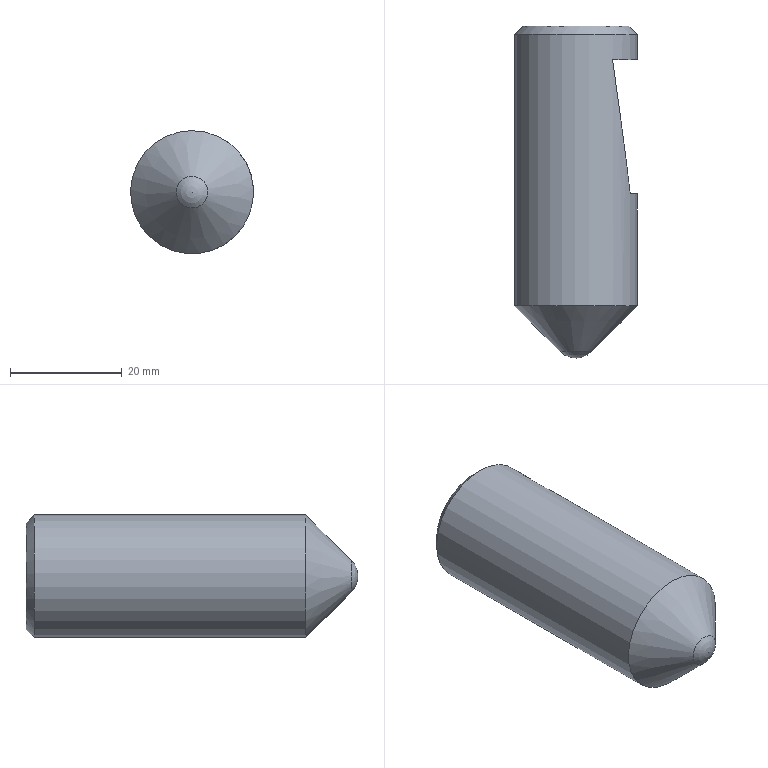Component | NX | LOCATING_SHAFT | 1 solid | 8 faces | box 22 x 59.34 x 22 mm | volume 18738 mm3 | plane 4 | cone 2 | cylinder 1 | sphere 1 | commonest cylinder face diameters 22 x1
STEP:
#1=CARTESIAN_POINT('',(0.,0.,0.));
#2=DIRECTION('',(0.,0.,1.));
#3=DIRECTION('',(1.,0.,0.));
#4=AXIS2_PLACEMENT_3D('',#1,#2,#3);
#5=CARTESIAN_POINT('',(-30.536,-43.411,2.847));
#6=VERTEX_POINT('',#5);
#7=CARTESIAN_POINT('',(-19.911,-43.411,-0.));
#8=DIRECTION('',(0.,-1.,0.));
#9=DIRECTION('',(-0.9659,0.,0.2588));
#10=AXIS2_PLACEMENT_3D('',#7,#8,#9);
#11=CIRCLE('',#10,11.);
#12=CARTESIAN_POINT('',(-19.911,-91.911,-0.));
#13=DIRECTION('',(0.,1.,0.));
#14=DIRECTION('',(-0.9659,0.,0.2588));
#15=AXIS2_PLACEMENT_3D('',#12,#13,#14);
#16=CYLINDRICAL_SURFACE('',#15,11.);
#17=CARTESIAN_POINT('',(6.283,48.5));
#18=DIRECTION('',(-1.,0.));
#19=VECTOR('',#18,1.);
#20=LINE('',#17,#19);
#21=(GEOMETRIC_REPRESENTATION_CONTEXT(2)PARAMETRIC_REPRESENTATION_CONTEXT()REPRESENTATION_CONTEXT('',''));
#22=DEFINITIONAL_REPRESENTATION('',(#20),#21);
#23=PCURVE('',#16,#22);
#24=CARTESIAN_POINT('',(-19.911,-41.911,-0.));
#25=DIRECTION('',(0.,-1.,0.));
#26=DIRECTION('',(0.9659,0.,-0.2588));
#27=AXIS2_PLACEMENT_3D('',#24,#25,#26);
#28=CONICAL_SURFACE('',#27,9.5,0.7854);
#29=CARTESIAN_POINT('',(3.142,1.5));
#30=DIRECTION('',(1.,0.));
#31=VECTOR('',#30,1.);
#32=LINE('',#29,#31);
#33=(GEOMETRIC_REPRESENTATION_CONTEXT(2)PARAMETRIC_REPRESENTATION_CONTEXT()REPRESENTATION_CONTEXT('',''));
#34=DEFINITIONAL_REPRESENTATION('',(#32),#33);
#35=PCURVE('',#28,#34);
#36=SURFACE_CURVE('',#11,(#23,#35),.PCURVE_S1.);
#37=EDGE_CURVE('',#6,#6,#36,.T.);
#38=ORIENTED_EDGE('',*,*,#37,.T.);
#39=CARTESIAN_POINT('',(-30.536,-91.911,2.847));
#40=VERTEX_POINT('',#39);
#41=CARTESIAN_POINT('',(-30.536,-91.911,2.847));
#42=CARTESIAN_POINT('',(-30.536,-43.411,2.847));
#43=B_SPLINE_CURVE_WITH_KNOTS('',1,(#41,#42),.UNSPECIFIED.,.F.,.F.,(2,2),(0.,48.5),.PIECEWISE_BEZIER_KNOTS.);
#44=CARTESIAN_POINT('',(0.,0.));
#45=DIRECTION('',(0.,1.));
#46=VECTOR('',#45,1.);
#47=LINE('',#44,#46);
#48=(GEOMETRIC_REPRESENTATION_CONTEXT(2)PARAMETRIC_REPRESENTATION_CONTEXT()REPRESENTATION_CONTEXT('',''));
#49=DEFINITIONAL_REPRESENTATION('',(#47),#48);
#50=PCURVE('',#16,#49);
#51=CARTESIAN_POINT('',(6.283,0.));
#52=DIRECTION('',(0.,1.));
#53=VECTOR('',#52,1.);
#54=LINE('',#51,#53);
#55=(GEOMETRIC_REPRESENTATION_CONTEXT(2)PARAMETRIC_REPRESENTATION_CONTEXT()REPRESENTATION_CONTEXT('',''));
#56=DEFINITIONAL_REPRESENTATION('',(#54),#55);
#57=PCURVE('',#16,#56);
#58=SEAM_CURVE('',#43,(#50,#57),.PCURVE_S1.);
#59=EDGE_CURVE('',#40,#6,#58,.T.);
#60=ORIENTED_EDGE('',*,*,#59,.F.);
#61=CARTESIAN_POINT('',(-19.911,-91.911,-0.));
#62=DIRECTION('',(0.,1.,0.));
#63=DIRECTION('',(-0.9659,0.,0.2588));
#64=AXIS2_PLACEMENT_3D('',#61,#62,#63);
#65=CIRCLE('',#64,11.);
#66=CARTESIAN_POINT('',(0.,0.));
#67=DIRECTION('',(1.,0.));
#68=VECTOR('',#67,1.);
#69=LINE('',#66,#68);
#70=(GEOMETRIC_REPRESENTATION_CONTEXT(2)PARAMETRIC_REPRESENTATION_CONTEXT()REPRESENTATION_CONTEXT('',''));
#71=DEFINITIONAL_REPRESENTATION('',(#69),#70);
#72=PCURVE('',#16,#71);
#73=CARTESIAN_POINT('',(-19.911,-91.911,-0.));
#74=DIRECTION('',(0.,1.,0.));
#75=DIRECTION('',(-0.9659,0.,0.2588));
#76=AXIS2_PLACEMENT_3D('',#73,#74,#75);
#77=CONICAL_SURFACE('',#76,11.,0.7854);
#78=CARTESIAN_POINT('',(0.,0.));
#79=DIRECTION('',(1.,0.));
#80=VECTOR('',#79,1.);
#81=LINE('',#78,#80);
#82=(GEOMETRIC_REPRESENTATION_CONTEXT(2)PARAMETRIC_REPRESENTATION_CONTEXT()REPRESENTATION_CONTEXT('',''));
#83=DEFINITIONAL_REPRESENTATION('',(#81),#82);
#84=PCURVE('',#77,#83);
#85=SURFACE_CURVE('',#65,(#72,#84),.PCURVE_S1.);
#86=EDGE_CURVE('',#40,#40,#85,.T.);
#87=ORIENTED_EDGE('',*,*,#86,.T.);
#88=ORIENTED_EDGE('',*,*,#59,.T.);
#89=EDGE_LOOP('',(#38,#60,#87,#88));
#90=FACE_BOUND('',#89,.T.);
#91=CARTESIAN_POINT('',(-13.395,-47.911,8.863));
#92=VERTEX_POINT('',#91);
#93=CARTESIAN_POINT('',(-18.699,-47.911,-10.933));
#94=VERTEX_POINT('',#93);
#95=CARTESIAN_POINT('',(-19.911,-47.911,-0.));
#96=DIRECTION('',(0.,1.,0.));
#97=DIRECTION('',(0.9659,0.,-0.2588));
#98=AXIS2_PLACEMENT_3D('',#95,#96,#97);
#99=CIRCLE('',#98,11.);
#100=CARTESIAN_POINT('',(-3.142,44.));
#101=DIRECTION('',(1.,0.));
#102=VECTOR('',#101,1.);
#103=LINE('',#100,#102);
#104=(GEOMETRIC_REPRESENTATION_CONTEXT(2)PARAMETRIC_REPRESENTATION_CONTEXT()REPRESENTATION_CONTEXT('',''));
#105=DEFINITIONAL_REPRESENTATION('',(#103),#104);
#106=PCURVE('',#16,#105);
#107=CARTESIAN_POINT('',(-28.988,-47.911,-49.332));
#108=DIRECTION('',(0.,-1.,0.));
#109=DIRECTION('',(0.9659,0.,-0.2588));
#110=AXIS2_PLACEMENT_3D('',#107,#108,#109);
#111=PLANE('',#110);
#112=CARTESIAN_POINT('',(7.,50.));
#113=CARTESIAN_POINT('',(7.,30.947));
#114=CARTESIAN_POINT('',(-9.5,40.474));
#115=CARTESIAN_POINT('',(-26.,50.));
#116=CARTESIAN_POINT('',(-9.5,59.526));
#117=CARTESIAN_POINT('',(7.,69.053));
#118=CARTESIAN_POINT('',(7.,50.));
#119=(BOUNDED_CURVE()B_SPLINE_CURVE(2,(#112,#113,#114,#115,#116,#117,#118),.UNSPECIFIED.,.T.,.F.)B_SPLINE_CURVE_WITH_KNOTS((1,2,2,2,2,1),(-2.094,0.,2.094,4.189,6.283,8.378),.UNSPECIFIED.)CURVE()GEOMETRIC_REPRESENTATION_ITEM()RATIONAL_B_SPLINE_CURVE((1.,0.5,1.,0.5,1.,0.5,1.))REPRESENTATION_ITEM(''));
#120=(GEOMETRIC_REPRESENTATION_CONTEXT(2)PARAMETRIC_REPRESENTATION_CONTEXT()REPRESENTATION_CONTEXT('',''));
#121=DEFINITIONAL_REPRESENTATION('',(#119),#120);
#122=PCURVE('',#111,#121);
#123=SURFACE_CURVE('',#99,(#106,#122),.PCURVE_S1.);
#124=EDGE_CURVE('',#92,#94,#123,.T.);
#125=ORIENTED_EDGE('',*,*,#124,.T.);
#126=CARTESIAN_POINT('',(-14.138,-71.911,-9.363));
#127=VERTEX_POINT('',#126);
#128=CARTESIAN_POINT('',(-19.911,-23.911,-0.));
#129=DIRECTION('',(-0.9528,-0.1644,0.2553));
#130=DIRECTION('',(-0.1588,0.9864,0.04255));
#131=AXIS2_PLACEMENT_3D('',#128,#129,#130);
#132=ELLIPSE('',#131,66.91,11.);
#133=CARTESIAN_POINT('',(4.34,44.));
#134=CARTESIAN_POINT('',(4.334,43.588));
#135=CARTESIAN_POINT('',(4.32,42.768));
#136=CARTESIAN_POINT('',(4.3,41.547));
#137=CARTESIAN_POINT('',(4.28,40.337));
#138=CARTESIAN_POINT('',(4.26,39.138));
#139=CARTESIAN_POINT('',(4.24,37.951));
#140=CARTESIAN_POINT('',(4.22,36.776));
#141=CARTESIAN_POINT('',(4.2,35.614));
#142=CARTESIAN_POINT('',(4.179,34.464));
#143=CARTESIAN_POINT('',(4.159,33.328));
#144=CARTESIAN_POINT('',(4.139,32.207));
#145=CARTESIAN_POINT('',(4.119,31.099));
#146=CARTESIAN_POINT('',(4.099,30.007));
#147=CARTESIAN_POINT('',(4.079,28.93));
#148=CARTESIAN_POINT('',(4.059,27.869));
#149=CARTESIAN_POINT('',(4.039,26.824));
#150=CARTESIAN_POINT('',(4.019,25.795));
#151=CARTESIAN_POINT('',(3.999,24.784));
#152=CARTESIAN_POINT('',(3.978,23.79));
#153=CARTESIAN_POINT('',(3.958,22.814));
#154=CARTESIAN_POINT('',(3.938,21.856));
#155=CARTESIAN_POINT('',(3.918,20.917));
#156=CARTESIAN_POINT('',(3.905,20.303));
#157=CARTESIAN_POINT('',(3.898,20.));
#158=B_SPLINE_CURVE_WITH_KNOTS('',3,(#133,#134,#135,#136,#137,#138,#139,#140,#141,#142,#143,#144,#145,#146,#147,#148,#149,#150,#151,#152,#153,#154,#155,#156,#157),.UNSPECIFIED.,.F.,.F.,(4,1,1,1,1,1,1,1,1,1,1,1,1,1,1,1,1,1,1,1,1,1,4),(1.943,1.963,1.983,2.003,2.023,2.043,2.064,2.084,2.104,2.124,2.144,2.164,2.184,2.204,2.224,2.244,2.265,2.285,2.305,2.325,2.345,2.365,2.385),.QUASI_UNIFORM_KNOTS.);
#159=(GEOMETRIC_REPRESENTATION_CONTEXT(2)PARAMETRIC_REPRESENTATION_CONTEXT()REPRESENTATION_CONTEXT('',''));
#160=DEFINITIONAL_REPRESENTATION('',(#158),#159);
#161=PCURVE('',#16,#160);
#162=CARTESIAN_POINT('',(-25.125,-71.911,-50.367));
#163=DIRECTION('',(0.9528,0.1644,-0.2553));
#164=DIRECTION('',(-0.1588,0.9864,0.04255));
#165=AXIS2_PLACEMENT_3D('',#162,#163,#164);
#166=PLANE('',#165);
#167=CARTESIAN_POINT('',(115.572,50.));
#168=CARTESIAN_POINT('',(115.572,30.947));
#169=CARTESIAN_POINT('',(15.207,40.474));
#170=CARTESIAN_POINT('',(-85.159,50.));
#171=CARTESIAN_POINT('',(15.207,59.526));
#172=CARTESIAN_POINT('',(115.572,69.053));
#173=CARTESIAN_POINT('',(115.572,50.));
#174=(BOUNDED_CURVE()B_SPLINE_CURVE(2,(#167,#168,#169,#170,#171,#172,#173),.UNSPECIFIED.,.T.,.F.)B_SPLINE_CURVE_WITH_KNOTS((1,2,2,2,2,1),(-2.094,0.,2.094,4.189,6.283,8.378),.UNSPECIFIED.)CURVE()GEOMETRIC_REPRESENTATION_ITEM()RATIONAL_B_SPLINE_CURVE((1.,0.5,1.,0.5,1.,0.5,1.))REPRESENTATION_ITEM(''));
#175=(GEOMETRIC_REPRESENTATION_CONTEXT(2)PARAMETRIC_REPRESENTATION_CONTEXT()REPRESENTATION_CONTEXT('',''));
#176=DEFINITIONAL_REPRESENTATION('',(#174),#175);
#177=PCURVE('',#166,#176);
#178=SURFACE_CURVE('',#132,(#161,#177),.PCURVE_S1.);
#179=EDGE_CURVE('',#94,#127,#178,.T.);
#180=ORIENTED_EDGE('',*,*,#179,.T.);
#181=CARTESIAN_POINT('',(-10.23,-71.911,5.222));
#182=VERTEX_POINT('',#181);
#183=CARTESIAN_POINT('',(-19.911,-71.911,-0.));
#184=DIRECTION('',(0.,-1.,0.));
#185=DIRECTION('',(-0.9659,0.,0.2588));
#186=AXIS2_PLACEMENT_3D('',#183,#184,#185);
#187=CIRCLE('',#186,11.);
#188=CARTESIAN_POINT('',(6.283,20.));
#189=DIRECTION('',(-1.,0.));
#190=VECTOR('',#189,1.);
#191=LINE('',#188,#190);
#192=(GEOMETRIC_REPRESENTATION_CONTEXT(2)PARAMETRIC_REPRESENTATION_CONTEXT()REPRESENTATION_CONTEXT('',''));
#193=DEFINITIONAL_REPRESENTATION('',(#191),#192);
#194=PCURVE('',#16,#193);
#195=CARTESIAN_POINT('',(-22.227,-71.911,-51.143));
#196=DIRECTION('',(0.,1.,0.));
#197=DIRECTION('',(-0.9659,0.,0.2588));
#198=AXIS2_PLACEMENT_3D('',#195,#196,#197);
#199=PLANE('',#198);
#200=CARTESIAN_POINT('',(22.,50.));
#201=CARTESIAN_POINT('',(22.,30.947));
#202=CARTESIAN_POINT('',(5.5,40.474));
#203=CARTESIAN_POINT('',(-11.,50.));
#204=CARTESIAN_POINT('',(5.5,59.526));
#205=CARTESIAN_POINT('',(22.,69.053));
#206=CARTESIAN_POINT('',(22.,50.));
#207=(BOUNDED_CURVE()B_SPLINE_CURVE(2,(#200,#201,#202,#203,#204,#205,#206),.UNSPECIFIED.,.T.,.F.)B_SPLINE_CURVE_WITH_KNOTS((1,2,2,2,2,1),(-2.094,0.,2.094,4.189,6.283,8.378),.UNSPECIFIED.)CURVE()GEOMETRIC_REPRESENTATION_ITEM()RATIONAL_B_SPLINE_CURVE((1.,0.5,1.,0.5,1.,0.5,1.))REPRESENTATION_ITEM(''));
#208=(GEOMETRIC_REPRESENTATION_CONTEXT(2)PARAMETRIC_REPRESENTATION_CONTEXT()REPRESENTATION_CONTEXT('',''));
#209=DEFINITIONAL_REPRESENTATION('',(#207),#208);
#210=PCURVE('',#199,#209);
#211=SURFACE_CURVE('',#187,(#194,#210),.PCURVE_S1.);
#212=EDGE_CURVE('',#127,#182,#211,.T.);
#213=ORIENTED_EDGE('',*,*,#212,.T.);
#214=CARTESIAN_POINT('',(-19.911,-23.911,-0.));
#215=DIRECTION('',(-0.9528,-0.1644,0.2553));
#216=DIRECTION('',(-0.1588,0.9864,0.04255));
#217=AXIS2_PLACEMENT_3D('',#214,#215,#216);
#218=ELLIPSE('',#217,66.91,11.);
#219=CARTESIAN_POINT('',(2.385,20.));
#220=CARTESIAN_POINT('',(2.378,20.303));
#221=CARTESIAN_POINT('',(2.365,20.917));
#222=CARTESIAN_POINT('',(2.345,21.856));
#223=CARTESIAN_POINT('',(2.325,22.814));
#224=CARTESIAN_POINT('',(2.305,23.79));
#225=CARTESIAN_POINT('',(2.285,24.784));
#226=CARTESIAN_POINT('',(2.265,25.795));
#227=CARTESIAN_POINT('',(2.244,26.824));
#228=CARTESIAN_POINT('',(2.224,27.869));
#229=CARTESIAN_POINT('',(2.204,28.93));
#230=CARTESIAN_POINT('',(2.184,30.007));
#231=CARTESIAN_POINT('',(2.164,31.099));
#232=CARTESIAN_POINT('',(2.144,32.207));
#233=CARTESIAN_POINT('',(2.124,33.328));
#234=CARTESIAN_POINT('',(2.104,34.464));
#235=CARTESIAN_POINT('',(2.084,35.614));
#236=CARTESIAN_POINT('',(2.064,36.776));
#237=CARTESIAN_POINT('',(2.043,37.951));
#238=CARTESIAN_POINT('',(2.023,39.138));
#239=CARTESIAN_POINT('',(2.003,40.337));
#240=CARTESIAN_POINT('',(1.983,41.547));
#241=CARTESIAN_POINT('',(1.963,42.768));
#242=CARTESIAN_POINT('',(1.95,43.588));
#243=CARTESIAN_POINT('',(1.943,44.));
#244=B_SPLINE_CURVE_WITH_KNOTS('',3,(#219,#220,#221,#222,#223,#224,#225,#226,#227,#228,#229,#230,#231,#232,#233,#234,#235,#236,#237,#238,#239,#240,#241,#242,#243),.UNSPECIFIED.,.F.,.F.,(4,1,1,1,1,1,1,1,1,1,1,1,1,1,1,1,1,1,1,1,1,1,4),(3.898,3.918,3.938,3.958,3.978,3.999,4.019,4.039,4.059,4.079,4.099,4.119,4.139,4.159,4.179,4.2,4.22,4.24,4.26,4.28,4.3,4.32,4.34),.QUASI_UNIFORM_KNOTS.);
#245=(GEOMETRIC_REPRESENTATION_CONTEXT(2)PARAMETRIC_REPRESENTATION_CONTEXT()REPRESENTATION_CONTEXT('',''));
#246=DEFINITIONAL_REPRESENTATION('',(#244),#245);
#247=PCURVE('',#16,#246);
#248=CARTESIAN_POINT('',(115.572,50.));
#249=CARTESIAN_POINT('',(115.572,30.947));
#250=CARTESIAN_POINT('',(15.207,40.474));
#251=CARTESIAN_POINT('',(-85.159,50.));
#252=CARTESIAN_POINT('',(15.207,59.526));
#253=CARTESIAN_POINT('',(115.572,69.053));
#254=CARTESIAN_POINT('',(115.572,50.));
#255=(BOUNDED_CURVE()B_SPLINE_CURVE(2,(#248,#249,#250,#251,#252,#253,#254),.UNSPECIFIED.,.T.,.F.)B_SPLINE_CURVE_WITH_KNOTS((1,2,2,2,2,1),(-2.094,0.,2.094,4.189,6.283,8.378),.UNSPECIFIED.)CURVE()GEOMETRIC_REPRESENTATION_ITEM()RATIONAL_B_SPLINE_CURVE((1.,0.5,1.,0.5,1.,0.5,1.))REPRESENTATION_ITEM(''));
#256=(GEOMETRIC_REPRESENTATION_CONTEXT(2)PARAMETRIC_REPRESENTATION_CONTEXT()REPRESENTATION_CONTEXT('',''));
#257=DEFINITIONAL_REPRESENTATION('',(#255),#256);
#258=PCURVE('',#166,#257);
#259=SURFACE_CURVE('',#218,(#247,#258),.PCURVE_S1.);
#260=EDGE_CURVE('',#182,#92,#259,.T.);
#261=ORIENTED_EDGE('',*,*,#260,.T.);
#262=EDGE_LOOP('',(#125,#180,#213,#261));
#263=FACE_BOUND('',#262,.T.);
#264=ADVANCED_FACE('',(#90,#263),#16,.T.);
#265=CARTESIAN_POINT('',(-29.087,-41.911,2.459));
#266=VERTEX_POINT('',#265);
#267=CARTESIAN_POINT('',(-19.911,-41.911,-0.));
#268=DIRECTION('',(0.,1.,0.));
#269=DIRECTION('',(-0.9659,0.,0.2588));
#270=AXIS2_PLACEMENT_3D('',#267,#268,#269);
#271=CIRCLE('',#270,9.5);
#272=CARTESIAN_POINT('',(-19.911,-41.911,-0.));
#273=DIRECTION('',(0.,1.,0.));
#274=DIRECTION('',(-0.9659,0.,0.2588));
#275=AXIS2_PLACEMENT_3D('',#272,#273,#274);
#276=PLANE('',#275);
#277=CARTESIAN_POINT('',(0.,0.));
#278=DIRECTION('',(1.,0.));
#279=AXIS2_PLACEMENT_2D('',#277,#278);
#280=CIRCLE('',#279,9.5);
#281=(GEOMETRIC_REPRESENTATION_CONTEXT(2)PARAMETRIC_REPRESENTATION_CONTEXT()REPRESENTATION_CONTEXT('',''));
#282=DEFINITIONAL_REPRESENTATION('',(#280),#281);
#283=PCURVE('',#276,#282);
#284=CARTESIAN_POINT('',(9.425,-0.));
#285=DIRECTION('',(-1.,0.));
#286=VECTOR('',#285,1.);
#287=LINE('',#284,#286);
#288=(GEOMETRIC_REPRESENTATION_CONTEXT(2)PARAMETRIC_REPRESENTATION_CONTEXT()REPRESENTATION_CONTEXT('',''));
#289=DEFINITIONAL_REPRESENTATION('',(#287),#288);
#290=PCURVE('',#28,#289);
#291=SURFACE_CURVE('',#271,(#283,#290),.PCURVE_S1.);
#292=EDGE_CURVE('',#266,#266,#291,.T.);
#293=ORIENTED_EDGE('',*,*,#292,.T.);
#294=EDGE_LOOP('',(#293));
#295=FACE_BOUND('',#294,.T.);
#296=ADVANCED_FACE('',(#295),#276,.T.);
#297=CARTESIAN_POINT('',(-22.643,-100.083,0.7321));
#298=VERTEX_POINT('',#297);
#299=CARTESIAN_POINT('',(-17.179,-100.083,-0.7321));
#300=VERTEX_POINT('',#299);
#301=CARTESIAN_POINT('',(-19.911,-100.083,-0.));
#302=DIRECTION('',(0.,1.,0.));
#303=DIRECTION('',(-0.9659,0.,0.2588));
#304=AXIS2_PLACEMENT_3D('',#301,#302,#303);
#305=CIRCLE('',#304,2.828);
#306=CARTESIAN_POINT('',(0.,-8.172));
#307=DIRECTION('',(1.,0.));
#308=VECTOR('',#307,1.);
#309=LINE('',#306,#308);
#310=(GEOMETRIC_REPRESENTATION_CONTEXT(2)PARAMETRIC_REPRESENTATION_CONTEXT()REPRESENTATION_CONTEXT('',''));
#311=DEFINITIONAL_REPRESENTATION('',(#309),#310);
#312=PCURVE('',#77,#311);
#313=CARTESIAN_POINT('',(-19.911,-97.254,-0.));
#314=DIRECTION('',(0.,1.,-0.));
#315=DIRECTION('',(0.9659,-0.,-0.2588));
#316=AXIS2_PLACEMENT_3D('',#313,#314,#315);
#317=SPHERICAL_SURFACE('',#316,4.);
#318=CARTESIAN_POINT('',(3.142,-0.7854));
#319=CARTESIAN_POINT('',(3.237,-0.7854));
#320=CARTESIAN_POINT('',(3.427,-0.7854));
#321=CARTESIAN_POINT('',(3.713,-0.7854));
#322=CARTESIAN_POINT('',(3.998,-0.7854));
#323=CARTESIAN_POINT('',(4.284,-0.7854));
#324=CARTESIAN_POINT('',(4.57,-0.7854));
#325=CARTESIAN_POINT('',(4.855,-0.7854));
#326=CARTESIAN_POINT('',(5.141,-0.7854));
#327=CARTESIAN_POINT('',(5.426,-0.7854));
#328=CARTESIAN_POINT('',(5.712,-0.7854));
#329=CARTESIAN_POINT('',(5.998,-0.7854));
#330=CARTESIAN_POINT('',(6.283,-0.7854));
#331=CARTESIAN_POINT('',(6.569,-0.7854));
#332=CARTESIAN_POINT('',(6.854,-0.7854));
#333=CARTESIAN_POINT('',(7.14,-0.7854));
#334=CARTESIAN_POINT('',(7.426,-0.7854));
#335=CARTESIAN_POINT('',(7.711,-0.7854));
#336=CARTESIAN_POINT('',(7.997,-0.7854));
#337=CARTESIAN_POINT('',(8.282,-0.7854));
#338=CARTESIAN_POINT('',(8.568,-0.7854));
#339=CARTESIAN_POINT('',(8.854,-0.7854));
#340=CARTESIAN_POINT('',(9.139,-0.7854));
#341=CARTESIAN_POINT('',(9.33,-0.7854));
#342=CARTESIAN_POINT('',(9.425,-0.7854));
#343=B_SPLINE_CURVE_WITH_KNOTS('',3,(#318,#319,#320,#321,#322,#323,#324,#325,#326,#327,#328,#329,#330,#331,#332,#333,#334,#335,#336,#337,#338,#339,#340,#341,#342),.UNSPECIFIED.,.F.,.F.,(4,1,1,1,1,1,1,1,1,1,1,1,1,1,1,1,1,1,1,1,1,1,4),(0.,0.2856,0.5712,0.8568,1.142,1.428,1.714,1.999,2.285,2.57,2.856,3.142,3.427,3.713,3.998,4.284,4.57,4.855,5.141,5.426,5.712,5.998,6.283),.QUASI_UNIFORM_KNOTS.);
#344=(GEOMETRIC_REPRESENTATION_CONTEXT(2)PARAMETRIC_REPRESENTATION_CONTEXT()REPRESENTATION_CONTEXT('',''));
#345=DEFINITIONAL_REPRESENTATION('',(#343),#344);
#346=PCURVE('',#317,#345);
#347=SURFACE_CURVE('',#305,(#312,#346),.PCURVE_S1.);
#348=EDGE_CURVE('',#298,#300,#347,.T.);
#349=ORIENTED_EDGE('',*,*,#348,.T.);
#350=CARTESIAN_POINT('',(-19.911,-100.083,-0.));
#351=DIRECTION('',(0.,1.,0.));
#352=DIRECTION('',(-0.9659,0.,0.2588));
#353=AXIS2_PLACEMENT_3D('',#350,#351,#352);
#354=CIRCLE('',#353,2.828);
#355=CARTESIAN_POINT('',(0.,-8.172));
#356=DIRECTION('',(1.,0.));
#357=VECTOR('',#356,1.);
#358=LINE('',#355,#357);
#359=(GEOMETRIC_REPRESENTATION_CONTEXT(2)PARAMETRIC_REPRESENTATION_CONTEXT()REPRESENTATION_CONTEXT('',''));
#360=DEFINITIONAL_REPRESENTATION('',(#358),#359);
#361=PCURVE('',#77,#360);
#362=CARTESIAN_POINT('',(-3.142,-0.7854));
#363=CARTESIAN_POINT('',(-3.046,-0.7854));
#364=CARTESIAN_POINT('',(-2.856,-0.7854));
#365=CARTESIAN_POINT('',(-2.57,-0.7854));
#366=CARTESIAN_POINT('',(-2.285,-0.7854));
#367=CARTESIAN_POINT('',(-1.999,-0.7854));
#368=CARTESIAN_POINT('',(-1.714,-0.7854));
#369=CARTESIAN_POINT('',(-1.428,-0.7854));
#370=CARTESIAN_POINT('',(-1.142,-0.7854));
#371=CARTESIAN_POINT('',(-0.8568,-0.7854));
#372=CARTESIAN_POINT('',(-0.5712,-0.7854));
#373=CARTESIAN_POINT('',(-0.2856,-0.7854));
#374=CARTESIAN_POINT('',(-0.,-0.7854));
#375=CARTESIAN_POINT('',(0.2856,-0.7854));
#376=CARTESIAN_POINT('',(0.5712,-0.7854));
#377=CARTESIAN_POINT('',(0.8568,-0.7854));
#378=CARTESIAN_POINT('',(1.142,-0.7854));
#379=CARTESIAN_POINT('',(1.428,-0.7854));
#380=CARTESIAN_POINT('',(1.714,-0.7854));
#381=CARTESIAN_POINT('',(1.999,-0.7854));
#382=CARTESIAN_POINT('',(2.285,-0.7854));
#383=CARTESIAN_POINT('',(2.57,-0.7854));
#384=CARTESIAN_POINT('',(2.856,-0.7854));
#385=CARTESIAN_POINT('',(3.046,-0.7854));
#386=CARTESIAN_POINT('',(3.142,-0.7854));
#387=B_SPLINE_CURVE_WITH_KNOTS('',3,(#362,#363,#364,#365,#366,#367,#368,#369,#370,#371,#372,#373,#374,#375,#376,#377,#378,#379,#380,#381,#382,#383,#384,#385,#386),.UNSPECIFIED.,.F.,.F.,(4,1,1,1,1,1,1,1,1,1,1,1,1,1,1,1,1,1,1,1,1,1,4),(0.,0.2856,0.5712,0.8568,1.142,1.428,1.714,1.999,2.285,2.57,2.856,3.142,3.427,3.713,3.998,4.284,4.57,4.855,5.141,5.426,5.712,5.998,6.283),.QUASI_UNIFORM_KNOTS.);
#388=(GEOMETRIC_REPRESENTATION_CONTEXT(2)PARAMETRIC_REPRESENTATION_CONTEXT()REPRESENTATION_CONTEXT('',''));
#389=DEFINITIONAL_REPRESENTATION('',(#387),#388);
#390=PCURVE('',#317,#389);
#391=SURFACE_CURVE('',#354,(#361,#390),.PCURVE_S1.);
#392=EDGE_CURVE('',#300,#298,#391,.T.);
#393=ORIENTED_EDGE('',*,*,#392,.T.);
#394=CARTESIAN_POINT('',(-22.643,-100.083,0.7321));
#395=CARTESIAN_POINT('',(-30.536,-91.911,2.847));
#396=B_SPLINE_CURVE_WITH_KNOTS('',1,(#394,#395),.UNSPECIFIED.,.F.,.F.,(2,2),(-11.556,0.),.PIECEWISE_BEZIER_KNOTS.);
#397=CARTESIAN_POINT('',(6.283,0.));
#398=DIRECTION('',(0.,1.));
#399=VECTOR('',#398,1.);
#400=LINE('',#397,#399);
#401=(GEOMETRIC_REPRESENTATION_CONTEXT(2)PARAMETRIC_REPRESENTATION_CONTEXT()REPRESENTATION_CONTEXT('',''));
#402=DEFINITIONAL_REPRESENTATION('',(#400),#401);
#403=PCURVE('',#77,#402);
#404=CARTESIAN_POINT('',(0.,0.));
#405=DIRECTION('',(0.,1.));
#406=VECTOR('',#405,1.);
#407=LINE('',#404,#406);
#408=(GEOMETRIC_REPRESENTATION_CONTEXT(2)PARAMETRIC_REPRESENTATION_CONTEXT()REPRESENTATION_CONTEXT('',''));
#409=DEFINITIONAL_REPRESENTATION('',(#407),#408);
#410=PCURVE('',#77,#409);
#411=SEAM_CURVE('',#396,(#403,#410),.PCURVE_S1.);
#412=EDGE_CURVE('',#298,#40,#411,.T.);
#413=ORIENTED_EDGE('',*,*,#412,.T.);
#414=ORIENTED_EDGE('',*,*,#86,.F.);
#415=ORIENTED_EDGE('',*,*,#412,.F.);
#416=EDGE_LOOP('',(#349,#393,#413,#414,#415));
#417=FACE_BOUND('',#416,.T.);
#418=ADVANCED_FACE('',(#417),#77,.T.);
#419=ORIENTED_EDGE('',*,*,#392,.F.);
#420=CARTESIAN_POINT('',(-19.911,-101.254,-0.));
#421=VERTEX_POINT('',#420);
#422=CARTESIAN_POINT('',(-19.911,-101.254,-0.));
#423=CARTESIAN_POINT('',(-19.304,-101.254,-0.1626));
#424=CARTESIAN_POINT('',(-18.697,-101.131,-0.3252));
#425=CARTESIAN_POINT('',(-18.122,-100.884,-0.4795));
#426=CARTESIAN_POINT('',(-17.608,-100.527,-0.6171));
#427=CARTESIAN_POINT('',(-17.179,-100.083,-0.7321));
#428=B_SPLINE_CURVE_WITH_KNOTS('',5,(#422,#423,#424,#425,#426,#427),.UNSPECIFIED.,.F.,.F.,(6,6),(-1.571,-0.7854),.PIECEWISE_BEZIER_KNOTS.);
#429=CARTESIAN_POINT('',(0.,0.));
#430=DIRECTION('',(0.,1.));
#431=VECTOR('',#430,1.);
#432=LINE('',#429,#431);
#433=(GEOMETRIC_REPRESENTATION_CONTEXT(2)PARAMETRIC_REPRESENTATION_CONTEXT()REPRESENTATION_CONTEXT('',''));
#434=DEFINITIONAL_REPRESENTATION('',(#432),#433);
#435=PCURVE('',#317,#434);
#436=CARTESIAN_POINT('',(6.283,0.));
#437=DIRECTION('',(0.,1.));
#438=VECTOR('',#437,1.);
#439=LINE('',#436,#438);
#440=(GEOMETRIC_REPRESENTATION_CONTEXT(2)PARAMETRIC_REPRESENTATION_CONTEXT()REPRESENTATION_CONTEXT('',''));
#441=DEFINITIONAL_REPRESENTATION('',(#439),#440);
#442=PCURVE('',#317,#441);
#443=SEAM_CURVE('',#428,(#435,#442),.PCURVE_S1.);
#444=EDGE_CURVE('',#421,#300,#443,.T.);
#445=ORIENTED_EDGE('',*,*,#444,.F.);
#446=ORIENTED_EDGE('',*,*,#444,.T.);
#447=ORIENTED_EDGE('',*,*,#348,.F.);
#448=EDGE_LOOP('',(#419,#445,#446,#447));
#449=FACE_BOUND('',#448,.T.);
#450=ADVANCED_FACE('',(#449),#317,.T.);
#451=CARTESIAN_POINT('',(-25.125,-71.911,-50.367));
#452=DIRECTION('',(-0.2588,0.,-0.9659));
#453=VECTOR('',#452,1.);
#454=LINE('',#451,#453);
#455=CARTESIAN_POINT('',(3.,0.));
#456=DIRECTION('',(0.,-1.));
#457=VECTOR('',#456,1.);
#458=LINE('',#455,#457);
#459=(GEOMETRIC_REPRESENTATION_CONTEXT(2)PARAMETRIC_REPRESENTATION_CONTEXT()REPRESENTATION_CONTEXT('',''));
#460=DEFINITIONAL_REPRESENTATION('',(#458),#459);
#461=PCURVE('',#199,#460);
#462=CARTESIAN_POINT('',(0.,0.));
#463=DIRECTION('',(-0.,-1.));
#464=VECTOR('',#463,1.);
#465=LINE('',#462,#464);
#466=(GEOMETRIC_REPRESENTATION_CONTEXT(2)PARAMETRIC_REPRESENTATION_CONTEXT()REPRESENTATION_CONTEXT('',''));
#467=DEFINITIONAL_REPRESENTATION('',(#465),#466);
#468=PCURVE('',#166,#467);
#469=SURFACE_CURVE('',#454,(#461,#468),.PCURVE_S1.);
#470=EDGE_CURVE('',#182,#127,#469,.T.);
#471=ORIENTED_EDGE('',*,*,#470,.F.);
#472=ORIENTED_EDGE('',*,*,#212,.F.);
#473=EDGE_LOOP('',(#471,#472));
#474=FACE_BOUND('',#473,.T.);
#475=ADVANCED_FACE('',(#474),#199,.T.);
#476=CARTESIAN_POINT('',(-28.988,-47.911,-49.332));
#477=DIRECTION('',(-0.2588,0.,-0.9659));
#478=VECTOR('',#477,1.);
#479=LINE('',#476,#478);
#480=CARTESIAN_POINT('',(24.331,0.));
#481=DIRECTION('',(-0.,-1.));
#482=VECTOR('',#481,1.);
#483=LINE('',#480,#482);
#484=(GEOMETRIC_REPRESENTATION_CONTEXT(2)PARAMETRIC_REPRESENTATION_CONTEXT()REPRESENTATION_CONTEXT('',''));
#485=DEFINITIONAL_REPRESENTATION('',(#483),#484);
#486=PCURVE('',#166,#485);
#487=CARTESIAN_POINT('',(0.,0.));
#488=DIRECTION('',(0.,-1.));
#489=VECTOR('',#488,1.);
#490=LINE('',#487,#489);
#491=(GEOMETRIC_REPRESENTATION_CONTEXT(2)PARAMETRIC_REPRESENTATION_CONTEXT()REPRESENTATION_CONTEXT('',''));
#492=DEFINITIONAL_REPRESENTATION('',(#490),#491);
#493=PCURVE('',#111,#492);
#494=SURFACE_CURVE('',#479,(#486,#493),.PCURVE_S1.);
#495=EDGE_CURVE('',#92,#94,#494,.T.);
#496=ORIENTED_EDGE('',*,*,#495,.F.);
#497=ORIENTED_EDGE('',*,*,#260,.F.);
#498=ORIENTED_EDGE('',*,*,#470,.T.);
#499=ORIENTED_EDGE('',*,*,#179,.F.);
#500=EDGE_LOOP('',(#496,#497,#498,#499));
#501=FACE_BOUND('',#500,.T.);
#502=ADVANCED_FACE('',(#501),#166,.T.);
#503=ORIENTED_EDGE('',*,*,#124,.F.);
#504=ORIENTED_EDGE('',*,*,#495,.T.);
#505=EDGE_LOOP('',(#503,#504));
#506=FACE_BOUND('',#505,.T.);
#507=ADVANCED_FACE('',(#506),#111,.T.);
#508=ORIENTED_EDGE('',*,*,#37,.F.);
#509=CARTESIAN_POINT('',(-29.087,-41.911,2.459));
#510=CARTESIAN_POINT('',(-30.536,-43.411,2.847));
#511=B_SPLINE_CURVE_WITH_KNOTS('',1,(#509,#510),.UNSPECIFIED.,.F.,.F.,(2,2),(-0.,2.121),.PIECEWISE_BEZIER_KNOTS.);
#512=CARTESIAN_POINT('',(3.142,0.));
#513=DIRECTION('',(0.,1.));
#514=VECTOR('',#513,1.);
#515=LINE('',#512,#514);
#516=(GEOMETRIC_REPRESENTATION_CONTEXT(2)PARAMETRIC_REPRESENTATION_CONTEXT()REPRESENTATION_CONTEXT('',''));
#517=DEFINITIONAL_REPRESENTATION('',(#515),#516);
#518=PCURVE('',#28,#517);
#519=CARTESIAN_POINT('',(9.425,0.));
#520=DIRECTION('',(0.,1.));
#521=VECTOR('',#520,1.);
#522=LINE('',#519,#521);
#523=(GEOMETRIC_REPRESENTATION_CONTEXT(2)PARAMETRIC_REPRESENTATION_CONTEXT()REPRESENTATION_CONTEXT('',''));
#524=DEFINITIONAL_REPRESENTATION('',(#522),#523);
#525=PCURVE('',#28,#524);
#526=SEAM_CURVE('',#511,(#518,#525),.PCURVE_S1.);
#527=EDGE_CURVE('',#266,#6,#526,.T.);
#528=ORIENTED_EDGE('',*,*,#527,.F.);
#529=ORIENTED_EDGE('',*,*,#292,.F.);
#530=ORIENTED_EDGE('',*,*,#527,.T.);
#531=EDGE_LOOP('',(#508,#528,#529,#530));
#532=FACE_BOUND('',#531,.T.);
#533=ADVANCED_FACE('',(#532),#28,.T.);
#534=CLOSED_SHELL('',(#264,#296,#418,#450,#475,#502,#507,#533));
#535=MANIFOLD_SOLID_BREP('',#534);
#536=(LENGTH_UNIT()NAMED_UNIT(*)SI_UNIT(.MILLI.,.METRE.));
#537=UNCERTAINTY_MEASURE_WITH_UNIT(LENGTH_MEASURE(0.000005),#536,'','');
#538=(NAMED_UNIT(*)PLANE_ANGLE_UNIT()SI_UNIT($,.RADIAN.));
#539=(NAMED_UNIT(*)SI_UNIT($,.STERADIAN.)SOLID_ANGLE_UNIT());
#540=(GEOMETRIC_REPRESENTATION_CONTEXT(3)GLOBAL_UNCERTAINTY_ASSIGNED_CONTEXT((#537))GLOBAL_UNIT_ASSIGNED_CONTEXT((#536,#538,#539))REPRESENTATION_CONTEXT('',''));
#541=ADVANCED_BREP_SHAPE_REPRESENTATION('',(#4,#535),#540);